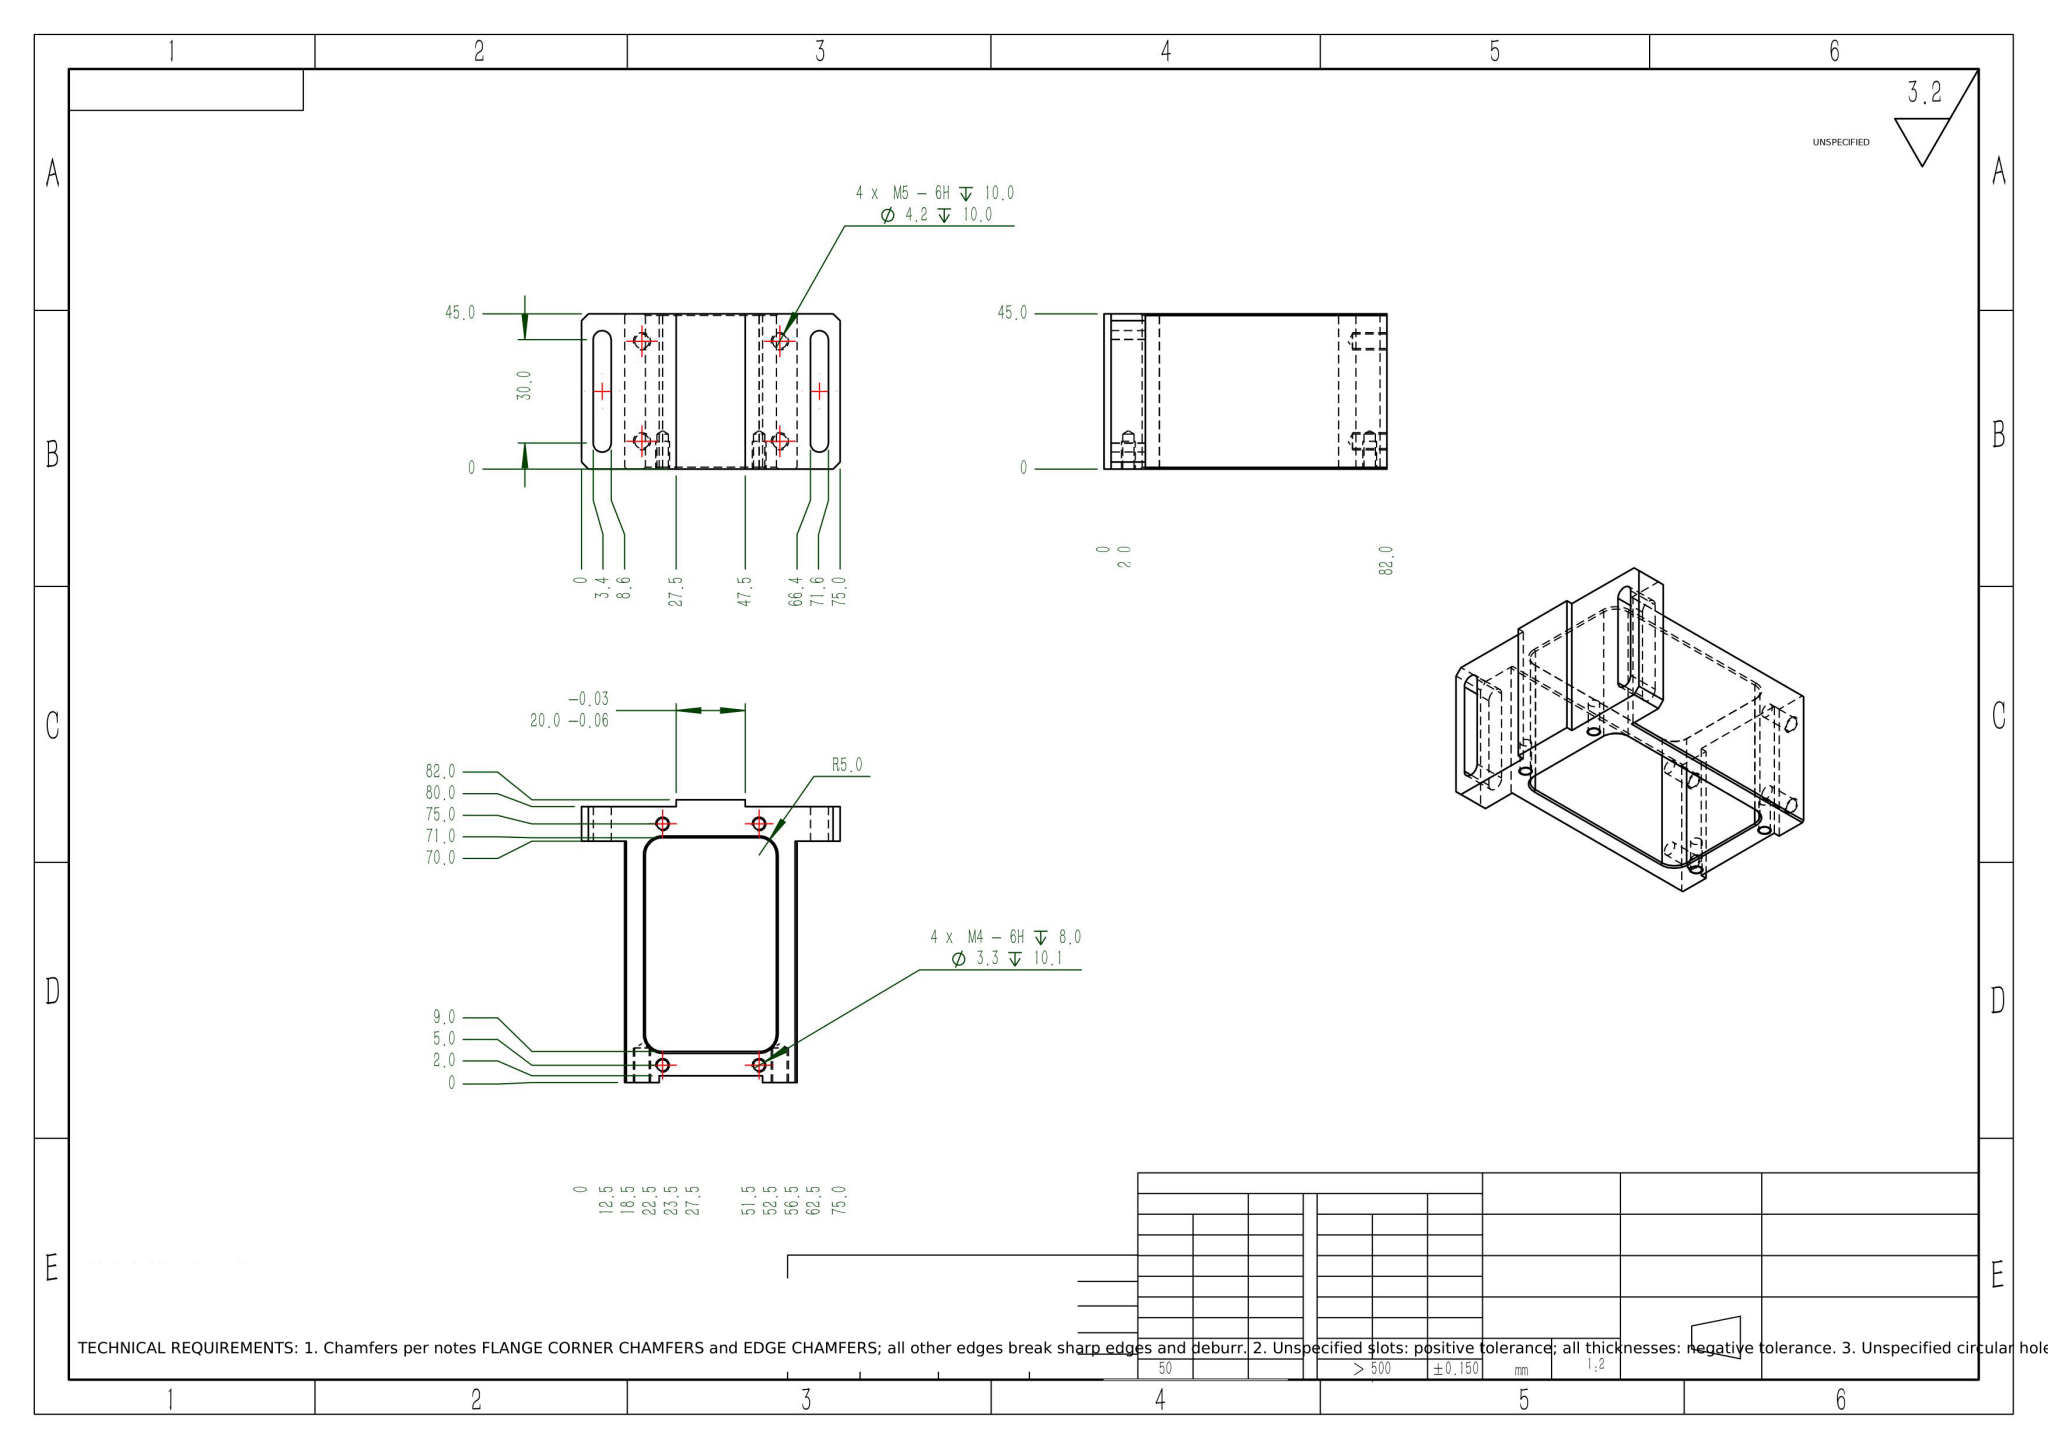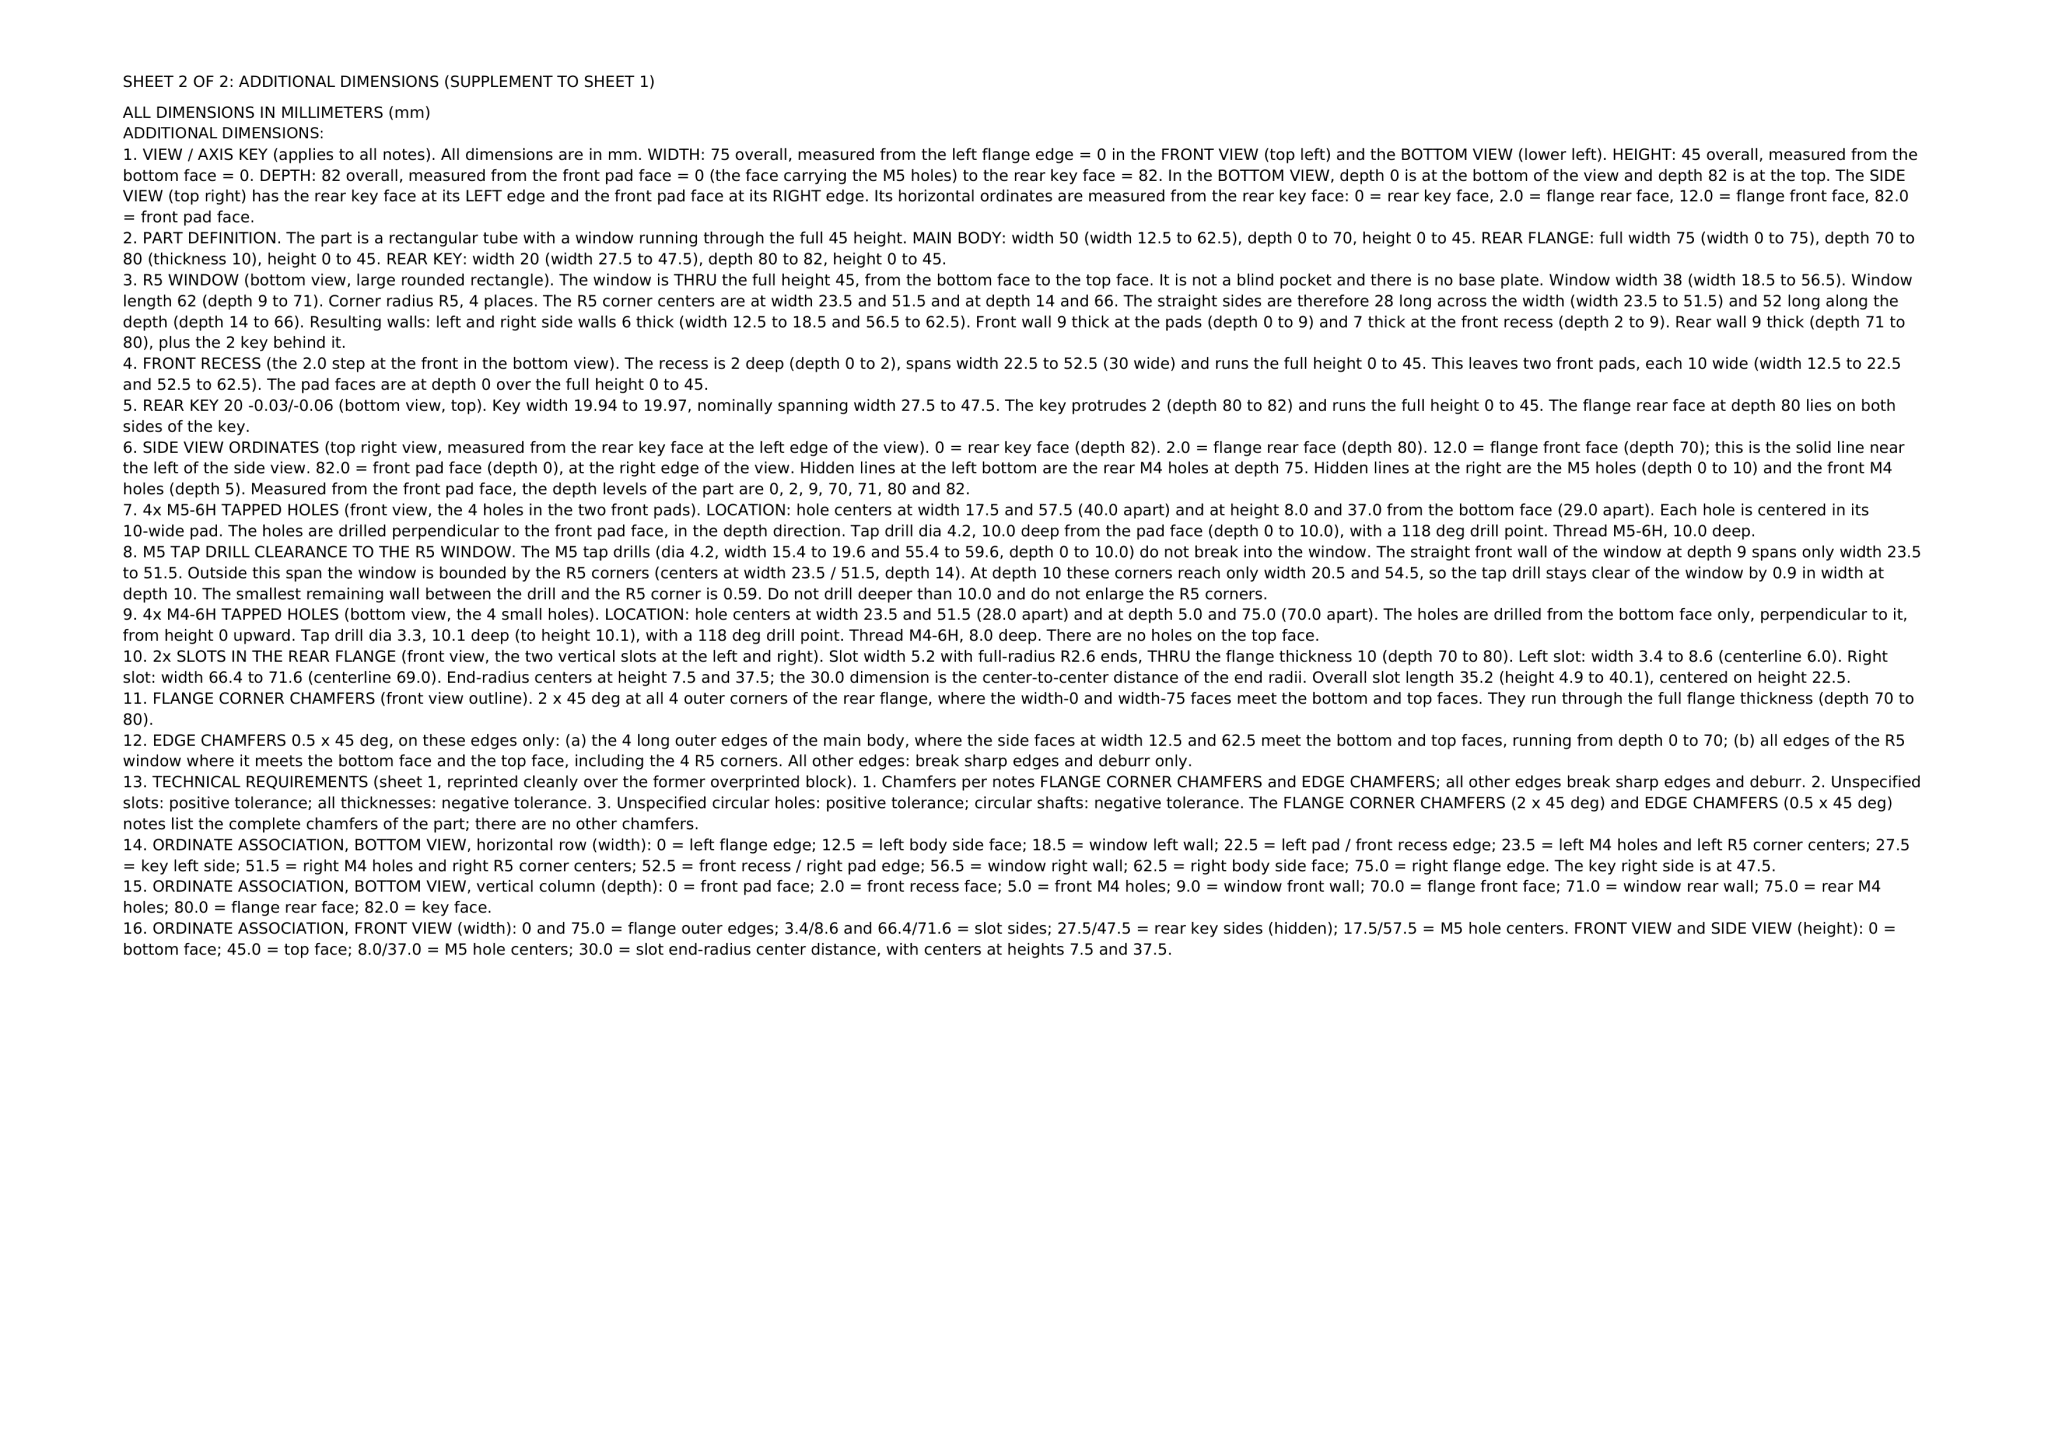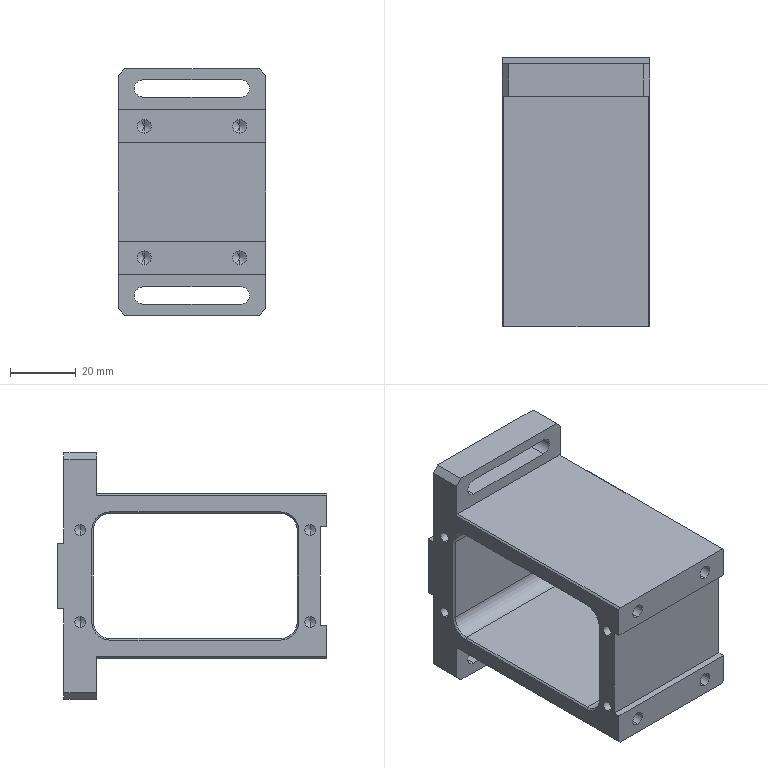Part | NX | mm | 1 solid | 92 faces | box 45 x 82 x 75 mm | volume 80654 mm3 | plane 42 | cylinder 26 | cone 24 | commonest cylinder face diameters 3.3 x8 4.2 x8 5.2 x6 10 x4